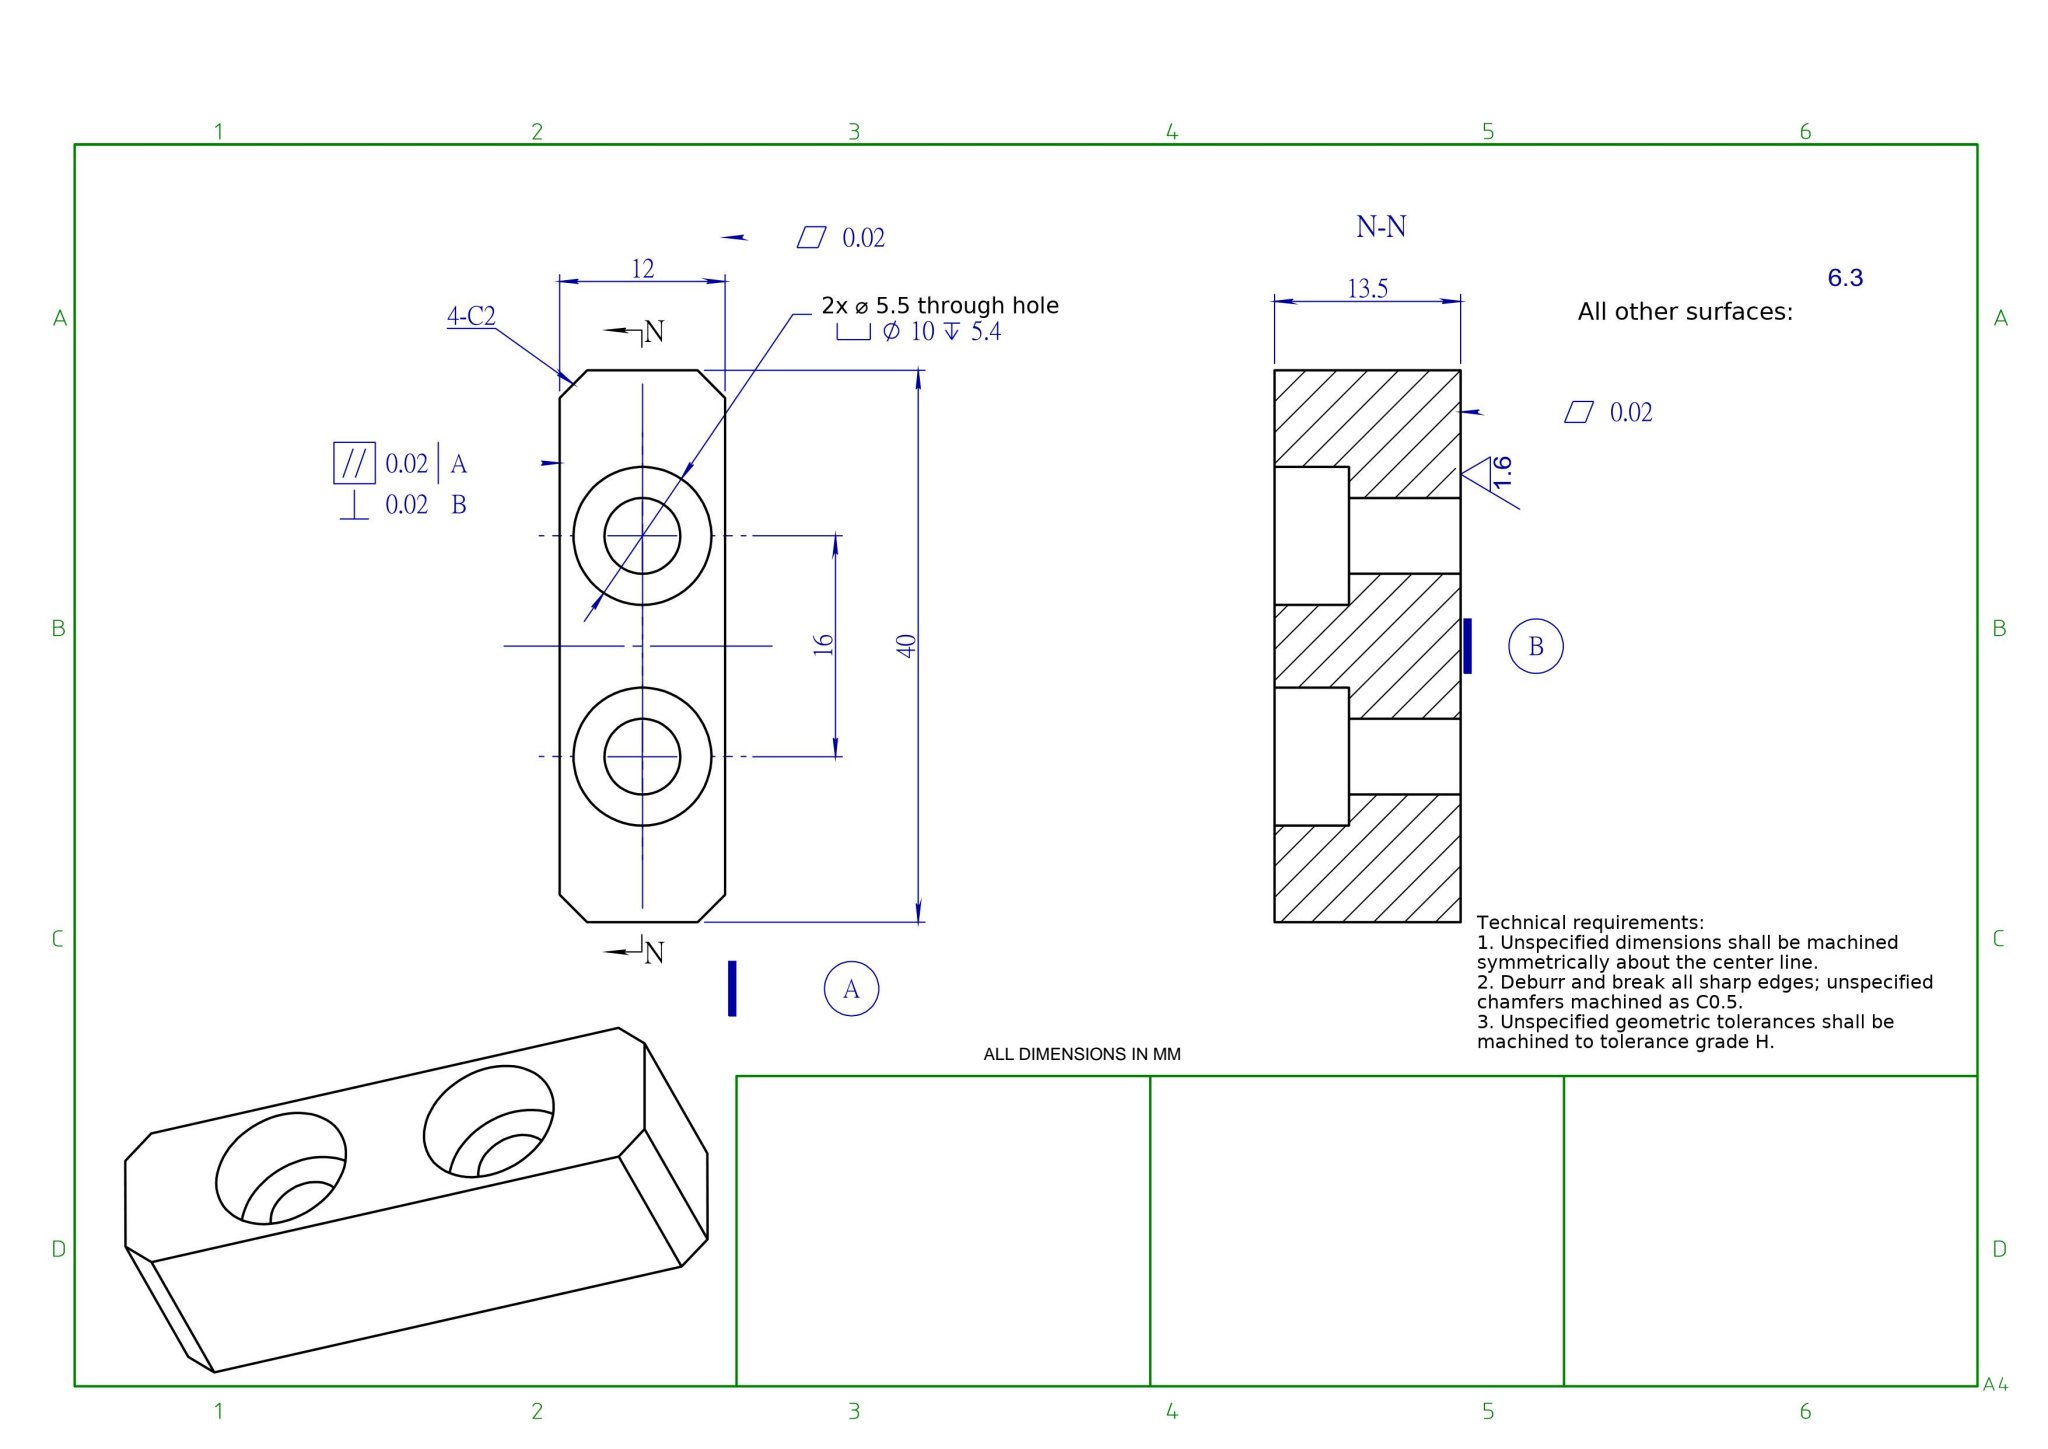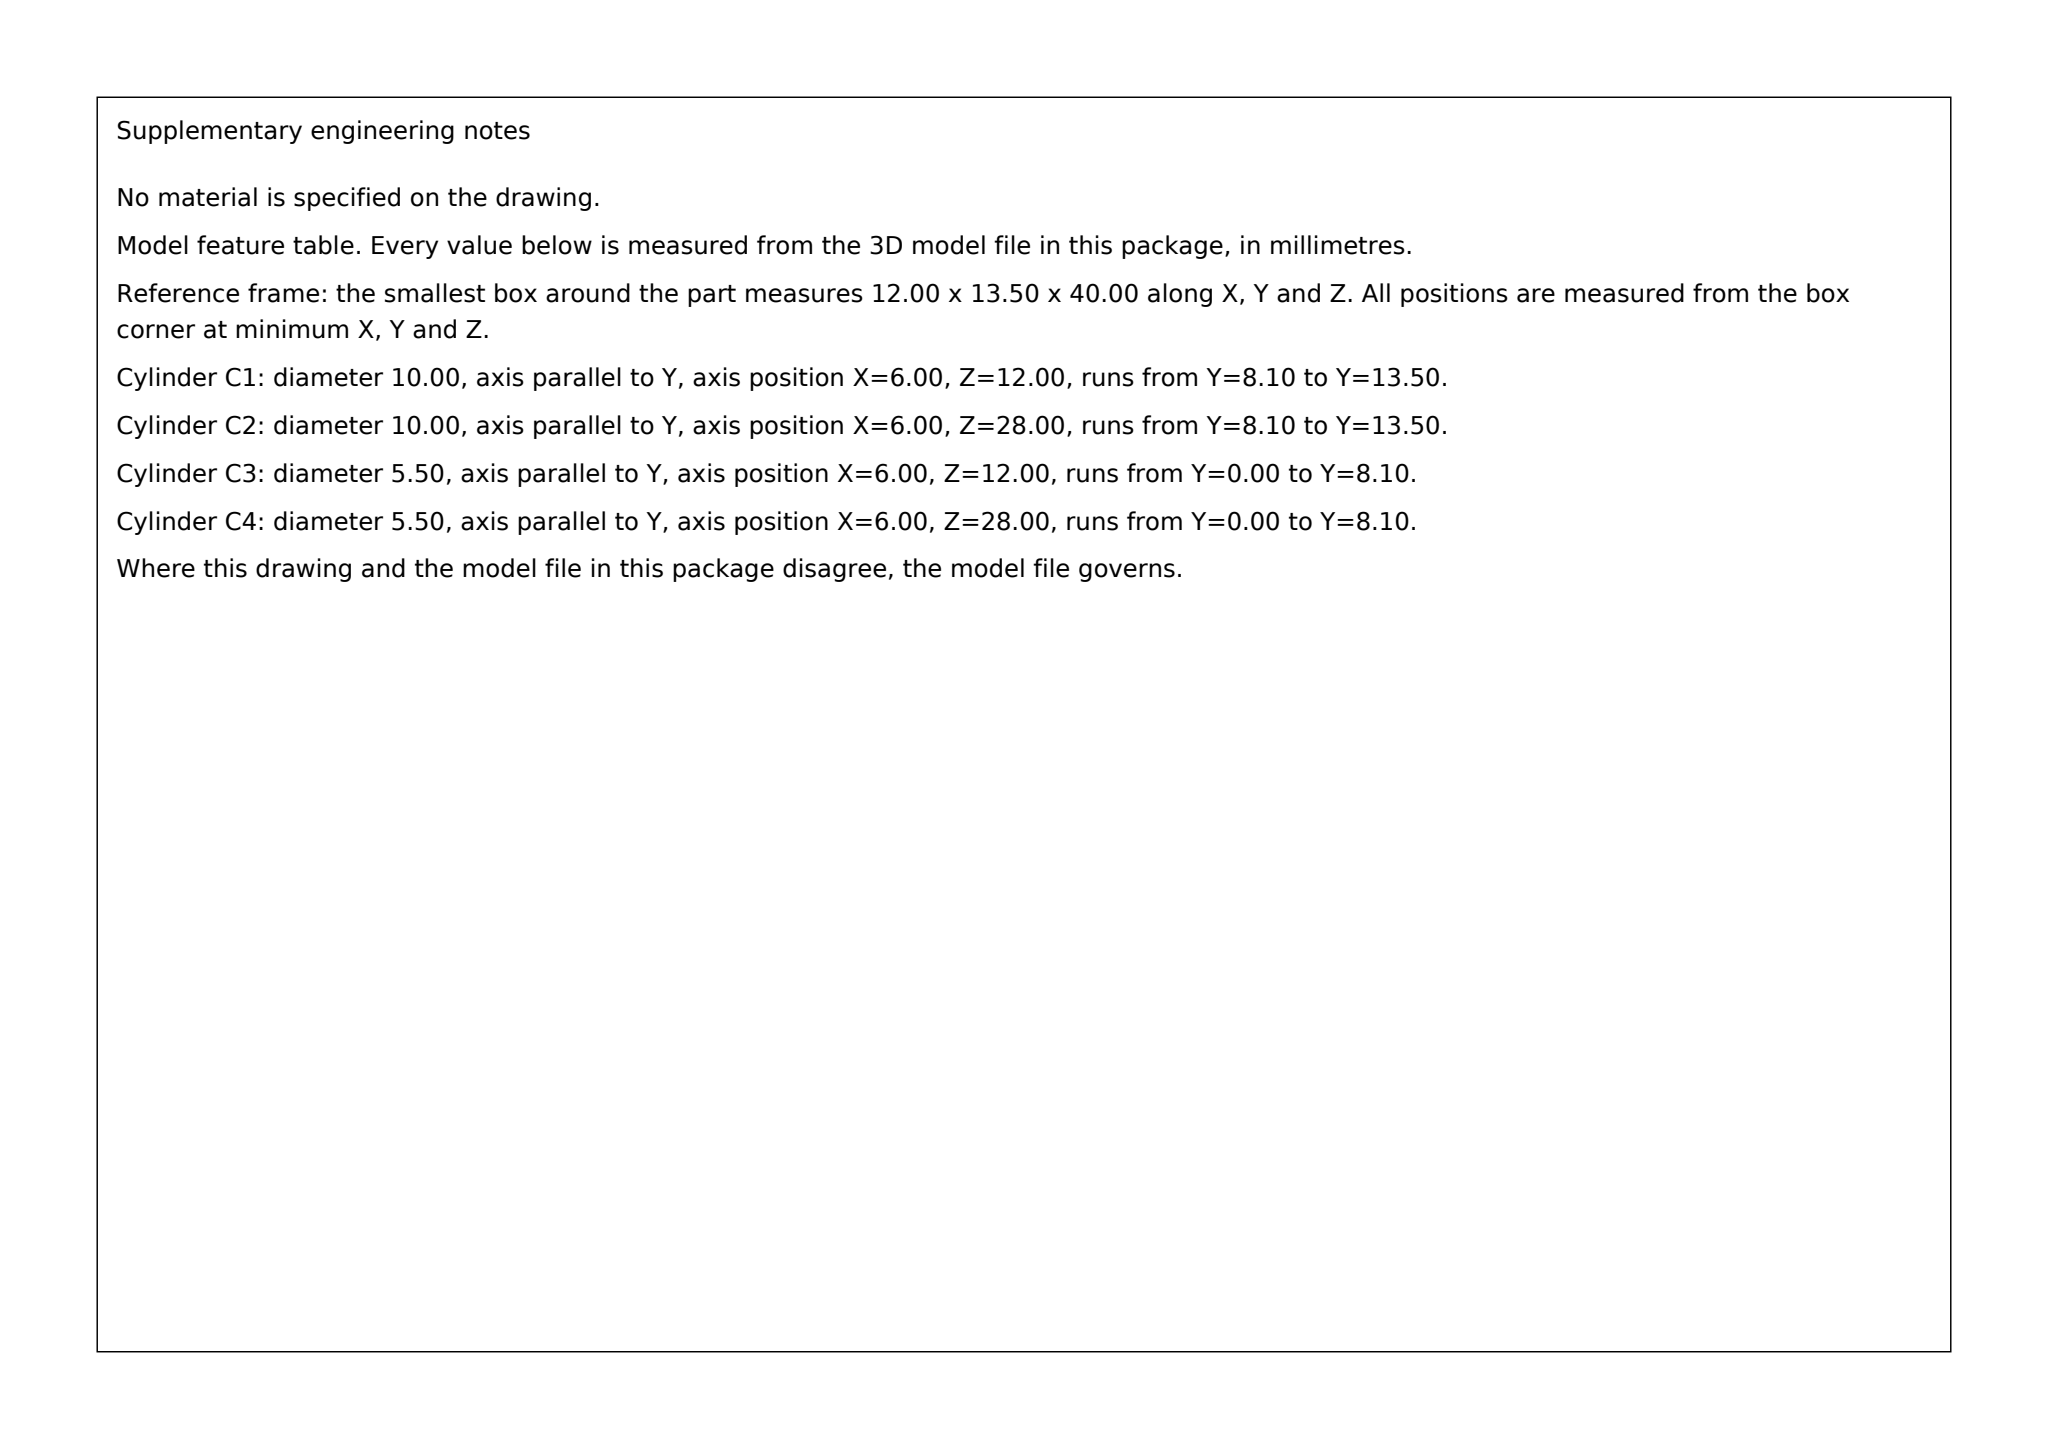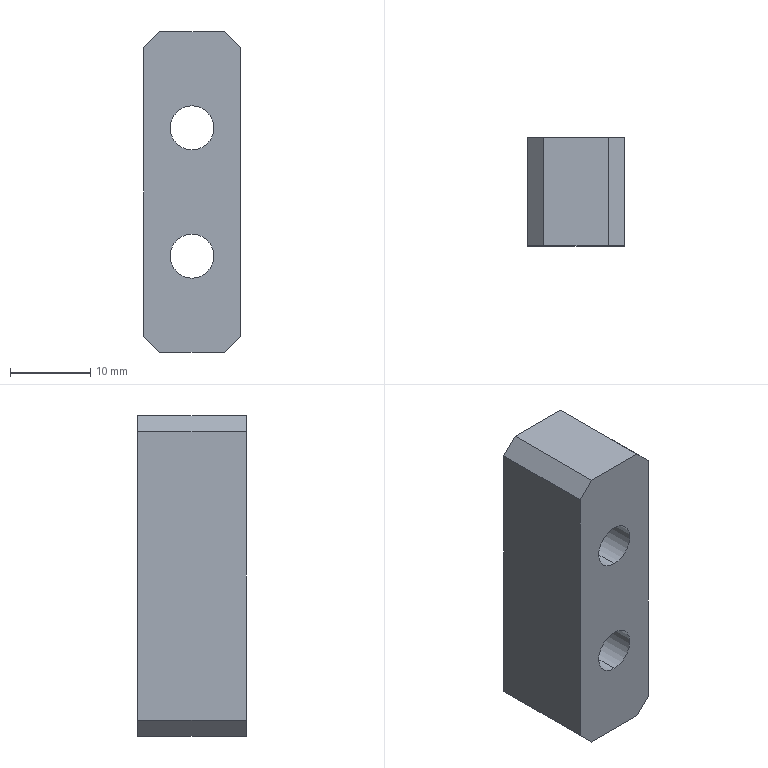Part | SolidWorks | mm | 1 solid | 20 faces | box 12 x 13.5 x 40 mm | volume 5139 mm3 | plane 12 | cylinder 8 | commonest cylinder face diameters 10 x4 5.5 x4
build123d program:
from build123d import *

# Parameters (mm, degrees)
SKETCH1_W                                            = 12
SKETCH1_H                                            = 13.5
EXTRUDE_THIN1_DEPTH                                  = 40
COUNTERBORE_FOR_M5_HEX_SOCKET_HEAD_CAP_S_D           = 5.5
COUNTERBORE_FOR_M5_HEX_SOCKET_HEAD_CAP_S_CBORE_D     = 10
COUNTERBORE_FOR_M5_HEX_SOCKET_HEAD_CAP_S_CBORE_DEPTH = 5.4
CHAMFER1_SIZE                                        = 2


with BuildPart() as part:
    # Sketch1 → Extrude-Thin1 (new body)
    with BuildSketch(Plane.XY):
        with Locations((-6, 6.75)):
            Rectangle(SKETCH1_W, SKETCH1_H)
    extrude(amount=EXTRUDE_THIN1_DEPTH)

    # Counterbore for M5 Hex Socket Head Cap S (through all)
    with Locations(Plane(origin=(0, 13.5, 0), x_dir=(1, 0, 0), z_dir=(0, 1, 0))):
        with Locations((-6, -12), (-6, -28)):
            CounterBoreHole(COUNTERBORE_FOR_M5_HEX_SOCKET_HEAD_CAP_S_D / 2, COUNTERBORE_FOR_M5_HEX_SOCKET_HEAD_CAP_S_CBORE_D / 2, COUNTERBORE_FOR_M5_HEX_SOCKET_HEAD_CAP_S_CBORE_DEPTH)

    # Chamfer1
    chamfer1_edges = [part.edges().sort_by_distance(p)[0] for p in [
        (0, 6.75, 40),
        (-12, 6.75, 40),
        (0, 6.75, 0),
        (-12, 6.75, 0),
    ]]
    chamfer(chamfer1_edges, length=CHAMFER1_SIZE)


solid = part.part